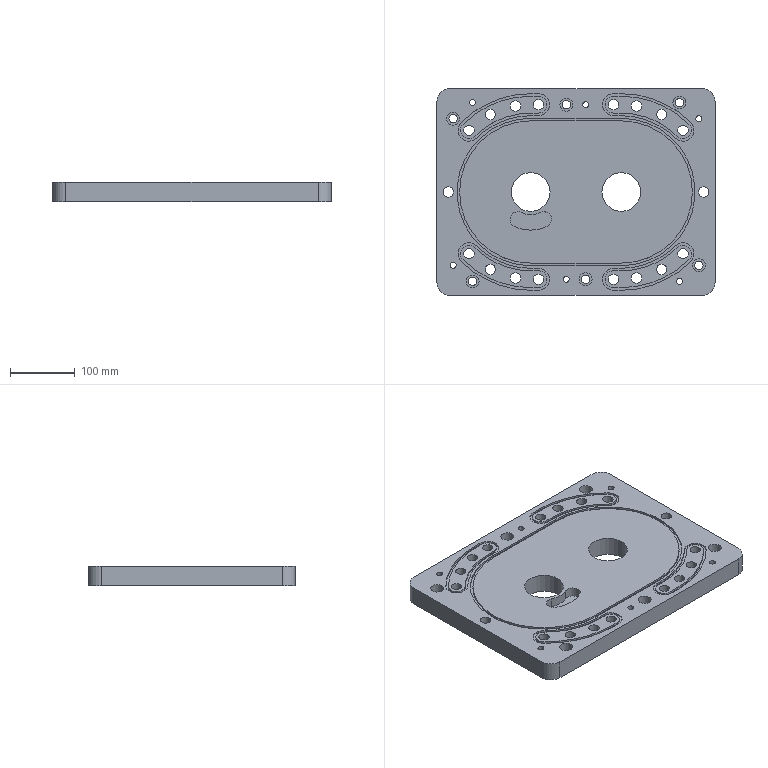CAM job | NX | mm | 3-axis | 1 set-up | 2 operations | part box 430 x 320 x 30
set-up 1
1. Cavity Milling | Mill Mill5 D16 | CAVITY_MILL | path 4835.818 mm | 9.904 min
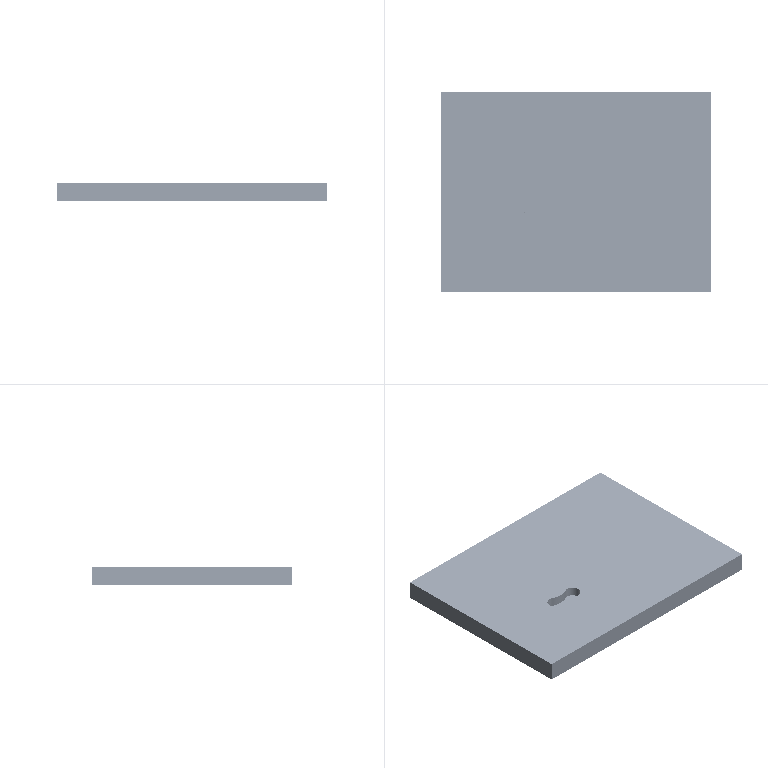2. Face Milling | Mill Mill5 D16 | FACE_MILLING | path 3668.405 mm | 9.051 min